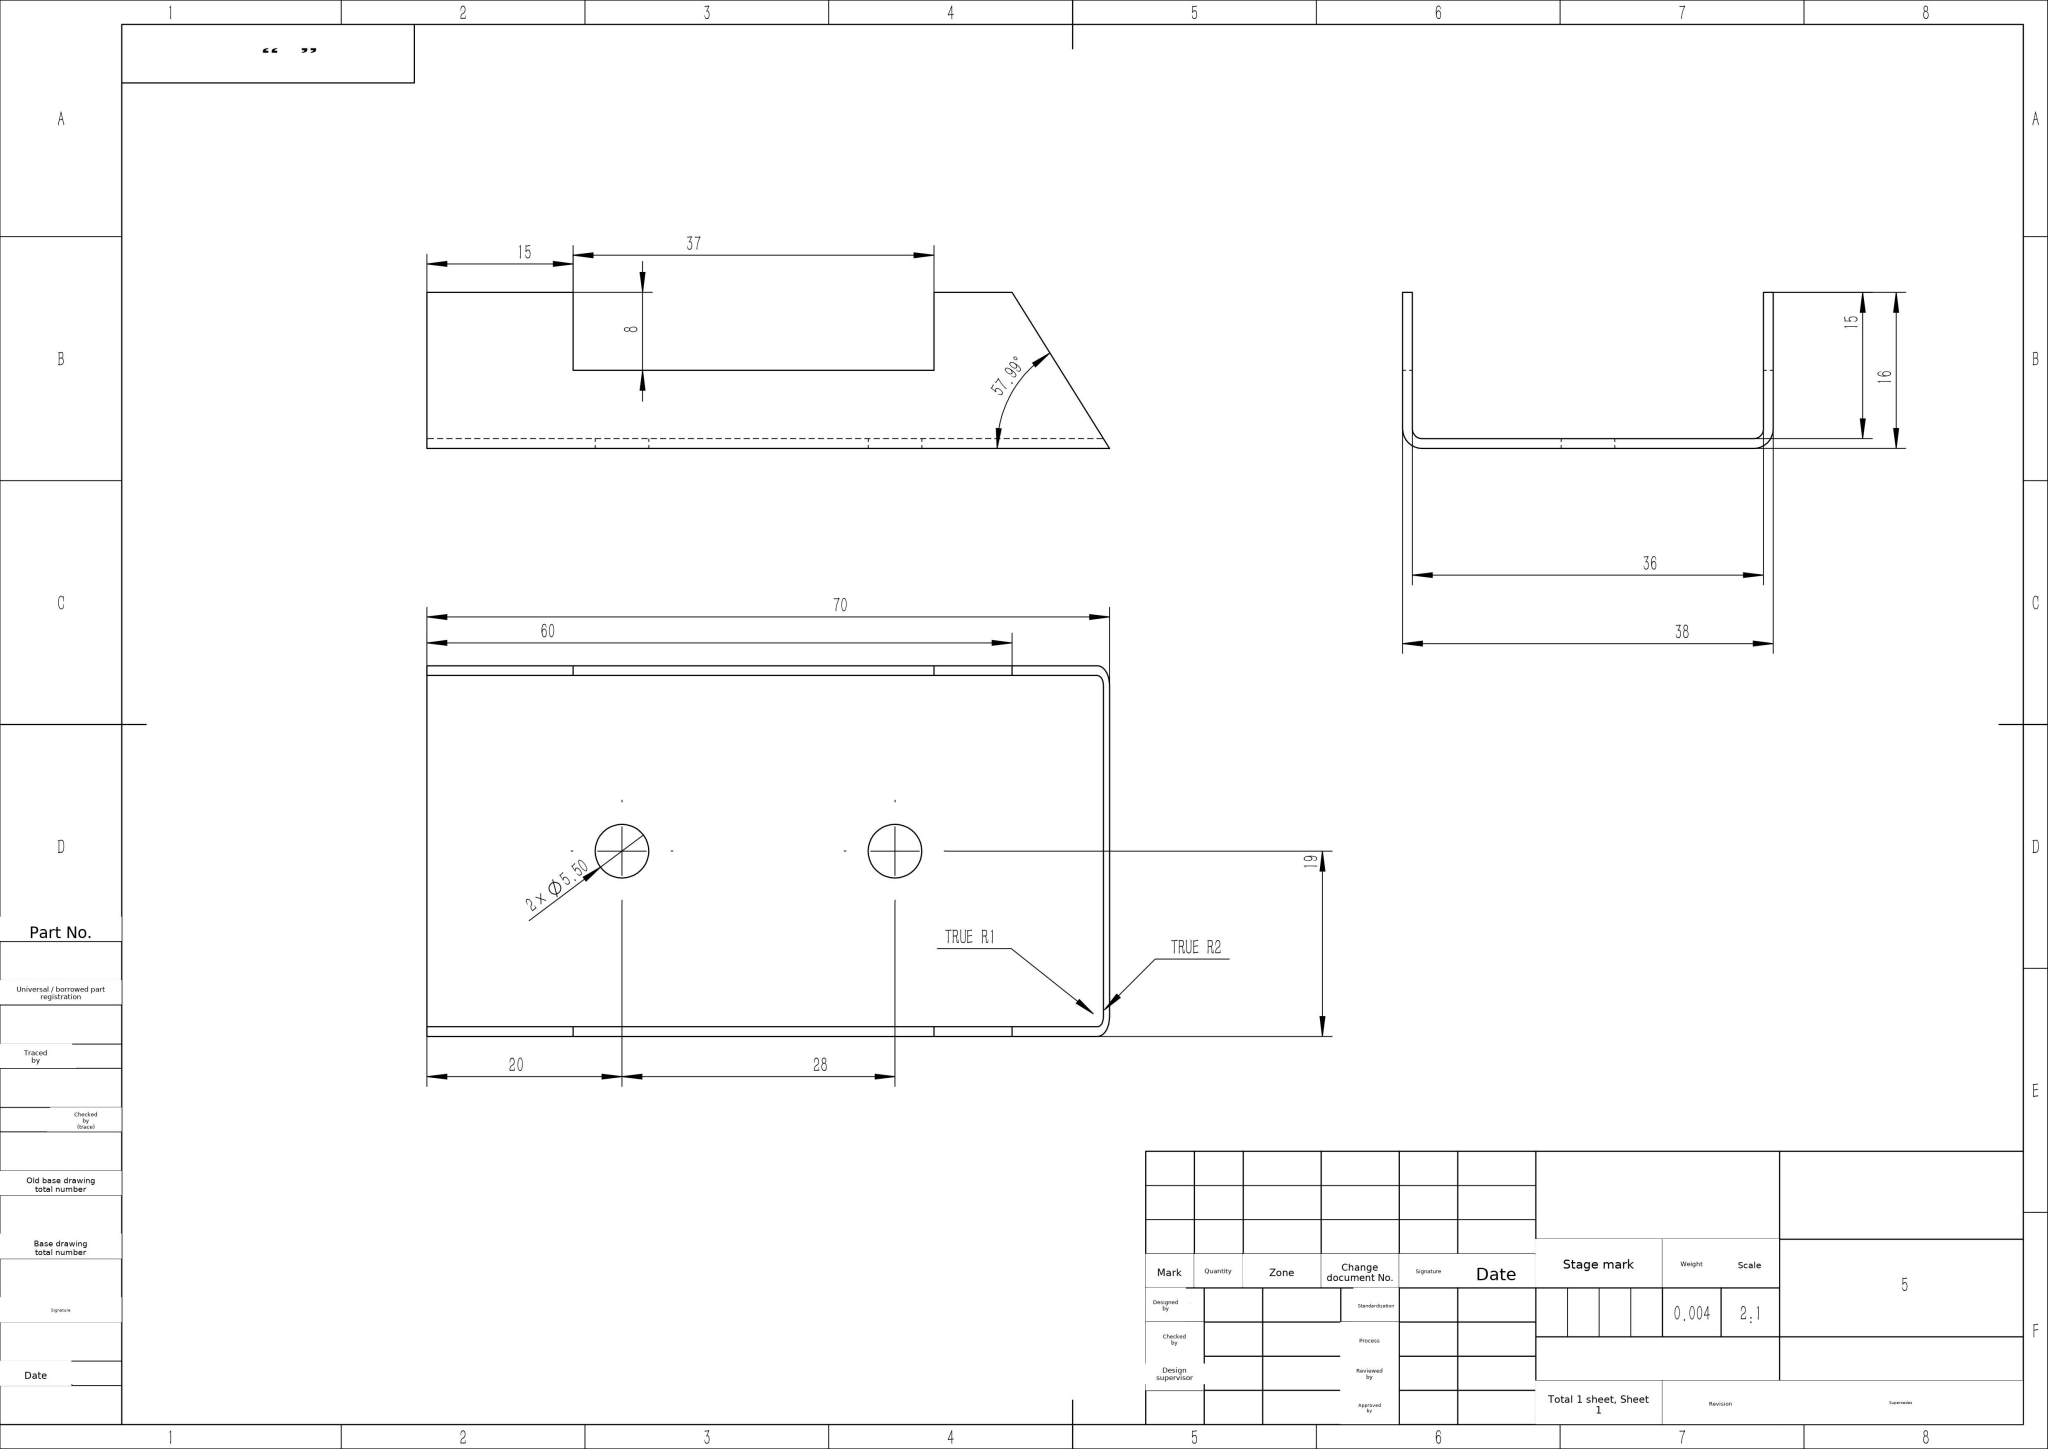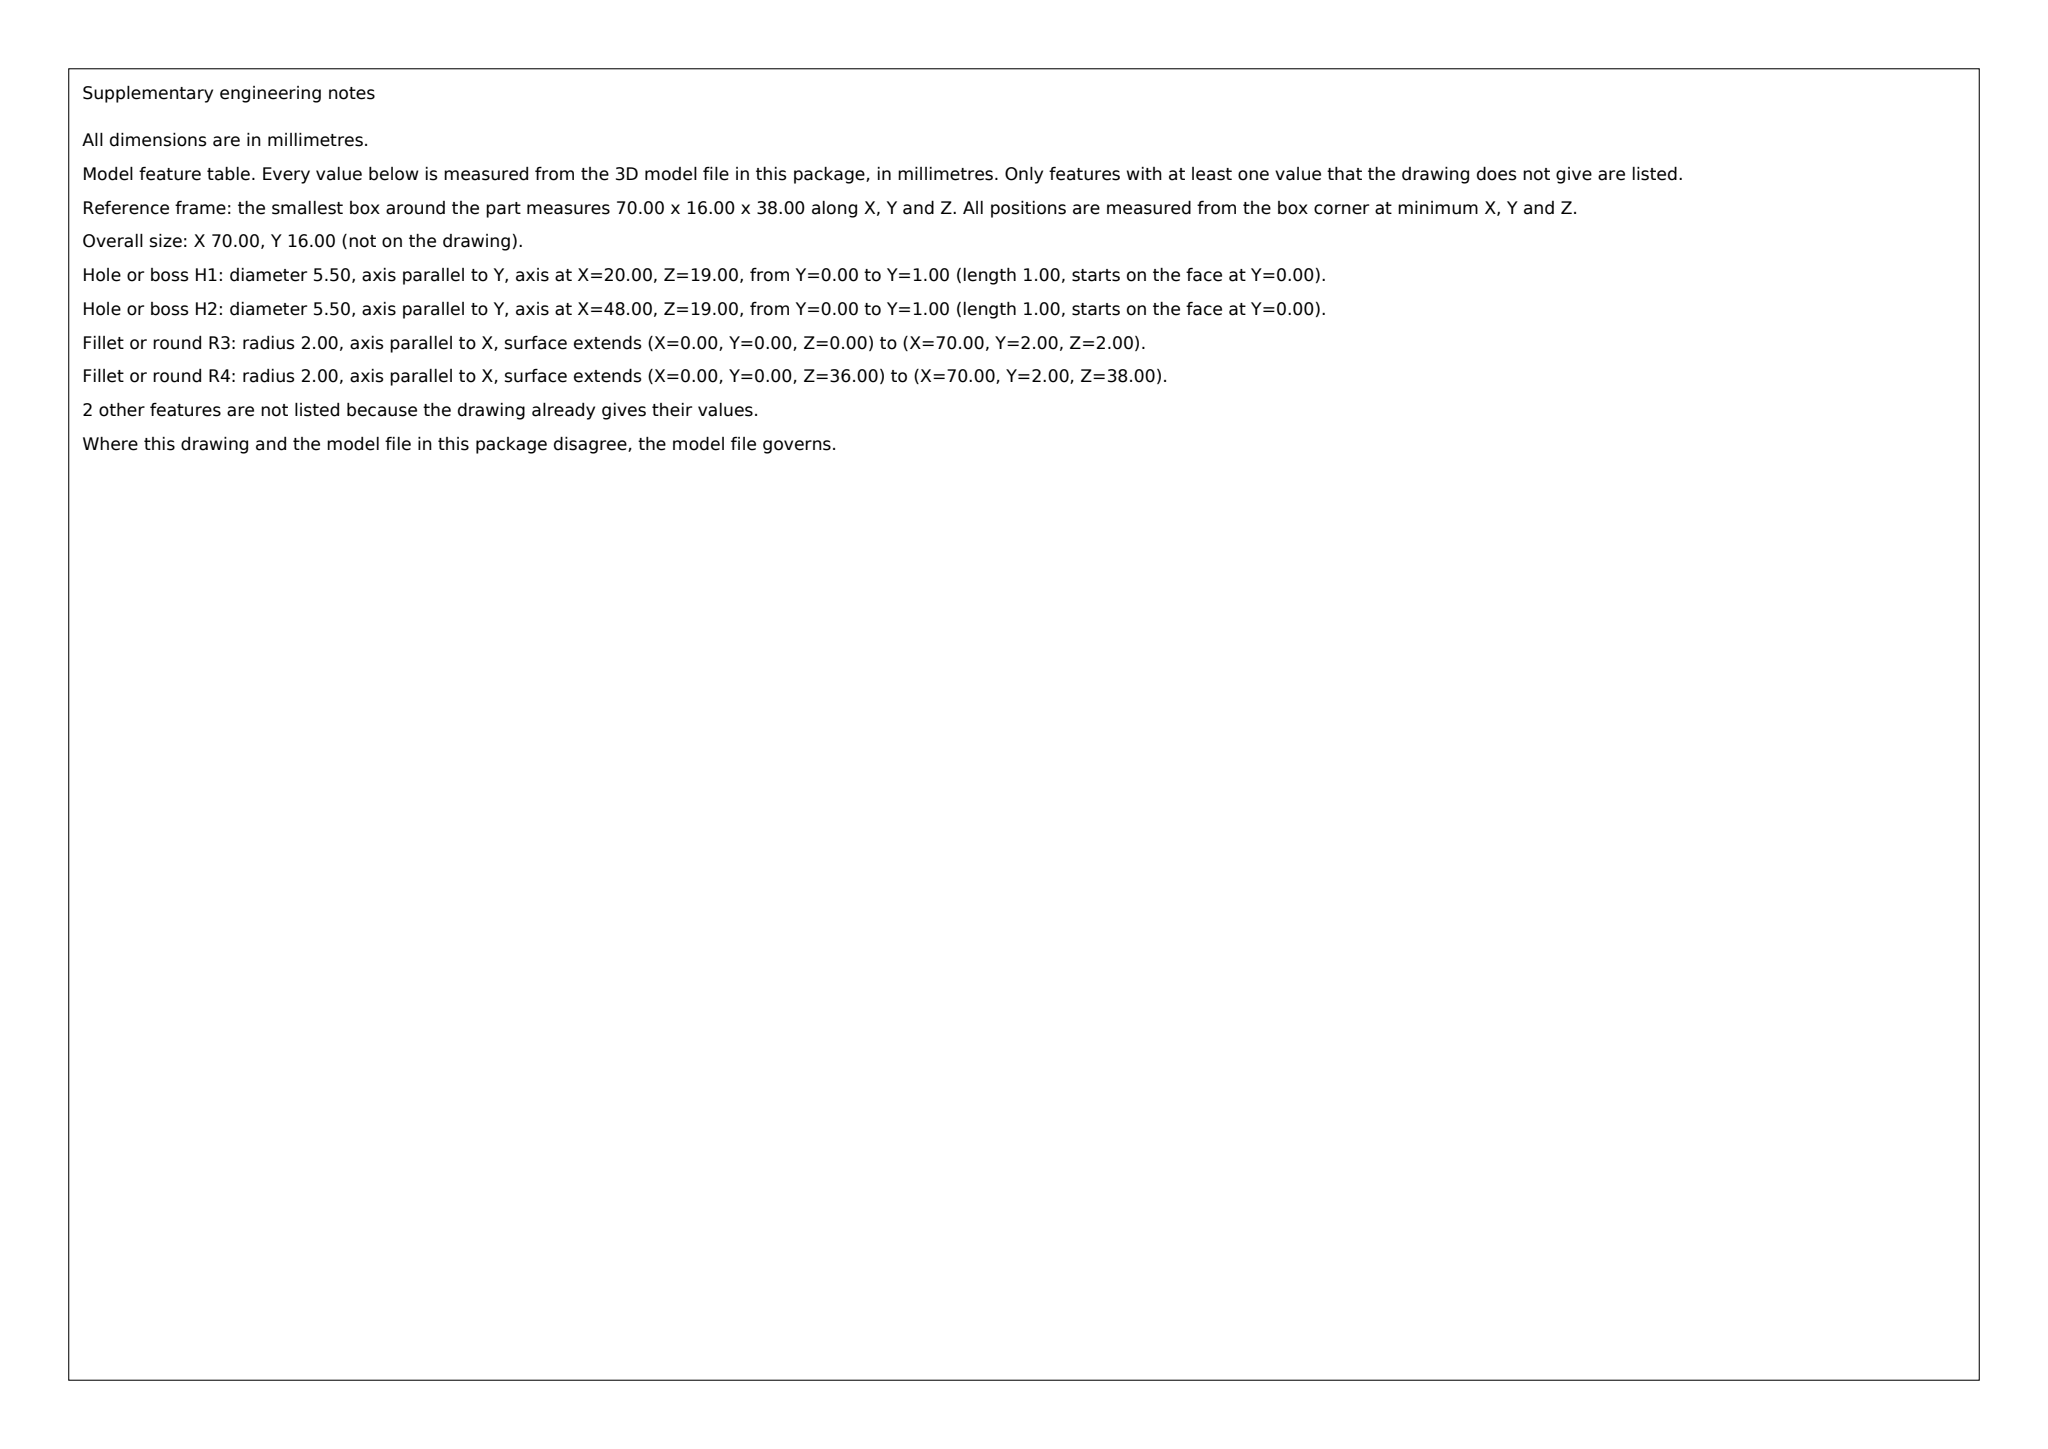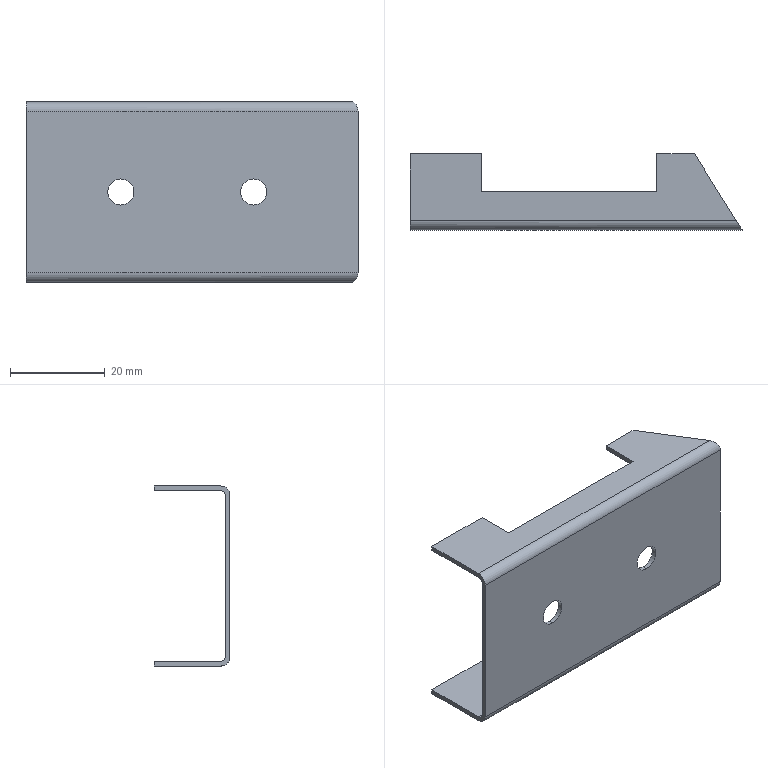Part | SolidWorks | mm | 1 solid | 26 faces | box 70 x 16 x 38 mm | volume 3859 mm3 | plane 18 | cylinder 8 | commonest cylinder face diameters 5.5 x4 2 x2 4 x2
build123d program:
from build123d import *

# Parameters (mm, degrees)
BOSS_EXTRUDE1_DEPTH = 70
FILLET1_R           = 1
FILLET2_R           = 2
SKETCH8_W           = 37
SKETCH8_H           = 9.122
CUT_EXTRUDE1_DEPTH  = 500
CUT_EXTRUDE2_DEPTH  = 500
SKETCH10_R          = 2.75
CUT_EXTRUDE3_DEPTH  = 500


with BuildPart() as part:
    # Sketch1 → Boss-Extrude1 (new body)
    with BuildSketch(Plane(origin=(0, 0, 0), x_dir=(0, 0, -1), z_dir=(1, 0, 0))):
        Polygon((-19, 0), (19, 0), (19, 16), (18, 16), (18, 1), (-18, 1), (-18, 16), (-19, 16), align=None)
    extrude(amount=BOSS_EXTRUDE1_DEPTH)

    # Fillet1
    fillet1_edges = [part.edges().sort_by_distance(p)[0] for p in [
        (35, 1, 18),
        (35, 1, -18),
    ]]
    fillet(fillet1_edges, radius=FILLET1_R)

    # Fillet2
    fillet2_edges = [part.edges().sort_by_distance(p)[0] for p in [
        (35, 0, -19),
        (35, 0, 19),
    ]]
    fillet(fillet2_edges, radius=FILLET2_R)

    # Sketch8 → Cut-Extrude1 (cut, symmetric)
    with BuildSketch(Plane.XY):
        with Locations((33.5, 12.561)):
            Rectangle(SKETCH8_W, SKETCH8_H)
    extrude(amount=CUT_EXTRUDE1_DEPTH, both=True, mode=Mode.SUBTRACT)

    # Sketch9 → Cut-Extrude2 (cut, symmetric)
    with BuildSketch(Plane.XY):
        Polygon((70, 0), (60, 16), (70, 16), align=None)
    extrude(amount=CUT_EXTRUDE2_DEPTH, both=True, mode=Mode.SUBTRACT)

    # Sketch10 → Cut-Extrude3 (cut, symmetric)
    with BuildSketch(Plane(origin=(0, 0, 0), x_dir=(1, 0, 0), z_dir=(0, 1, 0))):
        with Locations(Location((20, 0, 0), (0, 0, 270))):
            Circle(SKETCH10_R)
        with Locations(Location((48, 0, 0), (0, 0, 270))):
            Circle(SKETCH10_R)
    extrude(amount=CUT_EXTRUDE3_DEPTH, both=True, mode=Mode.SUBTRACT)


solid = part.part
STEP:
#1=CARTESIAN_POINT('',(20.,0.,-2.75));
#2=VERTEX_POINT('',#1);
#3=CARTESIAN_POINT('',(20.,-0.,2.75));
#4=VERTEX_POINT('',#3);
#5=CARTESIAN_POINT('',(20.,0.,0.));
#6=DIRECTION('',(0.,1.,0.));
#7=DIRECTION('',(0.,-0.,1.));
#8=AXIS2_PLACEMENT_3D('',#5,#6,#7);
#9=CIRCLE('',#8,2.75);
#10=EDGE_CURVE('',#2,#4,#9,.T.);
#11=ORIENTED_EDGE('',*,*,#10,.F.);
#12=CARTESIAN_POINT('',(20.,1.,-2.75));
#13=VERTEX_POINT('',#12);
#14=CARTESIAN_POINT('',(20.,-500.,-2.75));
#15=DIRECTION('',(0.,1.,0.));
#16=VECTOR('',#15,1000.);
#17=LINE('',#14,#16);
#18=EDGE_CURVE('',#2,#13,#17,.T.);
#19=ORIENTED_EDGE('',*,*,#18,.T.);
#20=CARTESIAN_POINT('',(20.,1.,2.75));
#21=VERTEX_POINT('',#20);
#22=CARTESIAN_POINT('',(20.,1.,0.));
#23=DIRECTION('',(0.,-1.,-0.));
#24=DIRECTION('',(0.,0.,-1.));
#25=AXIS2_PLACEMENT_3D('',#22,#23,#24);
#26=CIRCLE('',#25,2.75);
#27=EDGE_CURVE('',#21,#13,#26,.T.);
#28=ORIENTED_EDGE('',*,*,#27,.F.);
#29=CARTESIAN_POINT('',(20.,-500.,2.75));
#30=DIRECTION('',(0.,1.,0.));
#31=VECTOR('',#30,1000.);
#32=LINE('',#29,#31);
#33=EDGE_CURVE('',#4,#21,#32,.T.);
#34=ORIENTED_EDGE('',*,*,#33,.F.);
#35=EDGE_LOOP('',(#11,#19,#28,#34));
#36=FACE_OUTER_BOUND('',#35,.T.);
#37=CARTESIAN_POINT('',(20.,-500.,0.));
#38=DIRECTION('',(0.,1.,0.));
#39=DIRECTION('',(0.,0.,1.));
#40=AXIS2_PLACEMENT_3D('',#37,#38,#39);
#41=CYLINDRICAL_SURFACE('',#40,2.75);
#42=ADVANCED_FACE('',(#36),#41,.F.);
#43=CARTESIAN_POINT('',(48.,0.,-2.75));
#44=VERTEX_POINT('',#43);
#45=CARTESIAN_POINT('',(48.,-0.,2.75));
#46=VERTEX_POINT('',#45);
#47=CARTESIAN_POINT('',(48.,0.,0.));
#48=DIRECTION('',(0.,1.,0.));
#49=DIRECTION('',(0.,-0.,1.));
#50=AXIS2_PLACEMENT_3D('',#47,#48,#49);
#51=CIRCLE('',#50,2.75);
#52=EDGE_CURVE('',#44,#46,#51,.T.);
#53=ORIENTED_EDGE('',*,*,#52,.F.);
#54=CARTESIAN_POINT('',(48.,1.,-2.75));
#55=VERTEX_POINT('',#54);
#56=CARTESIAN_POINT('',(48.,-500.,-2.75));
#57=DIRECTION('',(0.,1.,0.));
#58=VECTOR('',#57,1000.);
#59=LINE('',#56,#58);
#60=EDGE_CURVE('',#44,#55,#59,.T.);
#61=ORIENTED_EDGE('',*,*,#60,.T.);
#62=CARTESIAN_POINT('',(48.,1.,2.75));
#63=VERTEX_POINT('',#62);
#64=CARTESIAN_POINT('',(48.,1.,0.));
#65=DIRECTION('',(0.,-1.,-0.));
#66=DIRECTION('',(0.,0.,-1.));
#67=AXIS2_PLACEMENT_3D('',#64,#65,#66);
#68=CIRCLE('',#67,2.75);
#69=EDGE_CURVE('',#63,#55,#68,.T.);
#70=ORIENTED_EDGE('',*,*,#69,.F.);
#71=CARTESIAN_POINT('',(48.,-500.,2.75));
#72=DIRECTION('',(0.,1.,0.));
#73=VECTOR('',#72,1000.);
#74=LINE('',#71,#73);
#75=EDGE_CURVE('',#46,#63,#74,.T.);
#76=ORIENTED_EDGE('',*,*,#75,.F.);
#77=EDGE_LOOP('',(#53,#61,#70,#76));
#78=FACE_OUTER_BOUND('',#77,.T.);
#79=CARTESIAN_POINT('',(48.,-500.,0.));
#80=DIRECTION('',(0.,1.,0.));
#81=DIRECTION('',(0.,0.,1.));
#82=AXIS2_PLACEMENT_3D('',#79,#80,#81);
#83=CYLINDRICAL_SURFACE('',#82,2.75);
#84=ADVANCED_FACE('',(#78),#83,.F.);
#85=CARTESIAN_POINT('',(15.,16.,18.));
#86=VERTEX_POINT('',#85);
#87=CARTESIAN_POINT('',(15.,16.,19.));
#88=VERTEX_POINT('',#87);
#89=CARTESIAN_POINT('',(15.,16.,19.));
#90=DIRECTION('',(0.,0.,1.));
#91=VECTOR('',#90,1000.);
#92=LINE('',#89,#91);
#93=EDGE_CURVE('',#86,#88,#92,.T.);
#94=ORIENTED_EDGE('',*,*,#93,.F.);
#95=CARTESIAN_POINT('',(0.,16.,18.));
#96=VERTEX_POINT('',#95);
#97=CARTESIAN_POINT('',(70.,16.,18.));
#98=DIRECTION('',(-1.,0.,0.));
#99=VECTOR('',#98,1000.);
#100=LINE('',#97,#99);
#101=EDGE_CURVE('',#86,#96,#100,.T.);
#102=ORIENTED_EDGE('',*,*,#101,.T.);
#103=CARTESIAN_POINT('',(0.,16.,19.));
#104=VERTEX_POINT('',#103);
#105=CARTESIAN_POINT('',(0.,16.,19.));
#106=DIRECTION('',(0.,0.,-1.));
#107=VECTOR('',#106,1000.);
#108=LINE('',#105,#107);
#109=EDGE_CURVE('',#104,#96,#108,.T.);
#110=ORIENTED_EDGE('',*,*,#109,.F.);
#111=CARTESIAN_POINT('',(70.,16.,19.));
#112=DIRECTION('',(-1.,0.,0.));
#113=VECTOR('',#112,1000.);
#114=LINE('',#111,#113);
#115=EDGE_CURVE('',#88,#104,#114,.T.);
#116=ORIENTED_EDGE('',*,*,#115,.F.);
#117=EDGE_LOOP('',(#94,#102,#110,#116));
#118=FACE_OUTER_BOUND('',#117,.T.);
#119=CARTESIAN_POINT('',(70.,16.,19.));
#120=DIRECTION('',(0.,1.,0.));
#121=DIRECTION('',(0.,0.,1.));
#122=AXIS2_PLACEMENT_3D('',#119,#120,#121);
#123=PLANE('',#122);
#124=ADVANCED_FACE('',(#118),#123,.T.);
#125=CARTESIAN_POINT('',(15.,16.,-18.));
#126=VERTEX_POINT('',#125);
#127=CARTESIAN_POINT('',(0.,16.,-18.));
#128=VERTEX_POINT('',#127);
#129=CARTESIAN_POINT('',(70.,16.,-18.));
#130=DIRECTION('',(-1.,0.,0.));
#131=VECTOR('',#130,1000.);
#132=LINE('',#129,#131);
#133=EDGE_CURVE('',#126,#128,#132,.T.);
#134=ORIENTED_EDGE('',*,*,#133,.F.);
#135=CARTESIAN_POINT('',(15.,16.,-19.));
#136=VERTEX_POINT('',#135);
#137=CARTESIAN_POINT('',(15.,16.,-19.));
#138=DIRECTION('',(0.,0.,-1.));
#139=VECTOR('',#138,1000.);
#140=LINE('',#137,#139);
#141=EDGE_CURVE('',#126,#136,#140,.T.);
#142=ORIENTED_EDGE('',*,*,#141,.T.);
#143=CARTESIAN_POINT('',(0.,16.,-19.));
#144=VERTEX_POINT('',#143);
#145=CARTESIAN_POINT('',(70.,16.,-19.));
#146=DIRECTION('',(-1.,0.,0.));
#147=VECTOR('',#146,1000.);
#148=LINE('',#145,#147);
#149=EDGE_CURVE('',#136,#144,#148,.T.);
#150=ORIENTED_EDGE('',*,*,#149,.T.);
#151=CARTESIAN_POINT('',(0.,16.,-19.));
#152=DIRECTION('',(0.,0.,1.));
#153=VECTOR('',#152,1000.);
#154=LINE('',#151,#153);
#155=EDGE_CURVE('',#144,#128,#154,.T.);
#156=ORIENTED_EDGE('',*,*,#155,.T.);
#157=EDGE_LOOP('',(#134,#142,#150,#156));
#158=FACE_OUTER_BOUND('',#157,.T.);
#159=CARTESIAN_POINT('',(70.,16.,-19.));
#160=DIRECTION('',(0.,-1.,0.));
#161=DIRECTION('',(0.,0.,-1.));
#162=AXIS2_PLACEMENT_3D('',#159,#160,#161);
#163=PLANE('',#162);
#164=ADVANCED_FACE('',(#158),#163,.F.);
#165=CARTESIAN_POINT('',(0.,2.,-18.));
#166=VERTEX_POINT('',#165);
#167=CARTESIAN_POINT('',(68.75,2.,-18.));
#168=VERTEX_POINT('',#167);
#169=CARTESIAN_POINT('',(70.,2.,-18.));
#170=DIRECTION('',(1.,0.,0.));
#171=VECTOR('',#170,1000.);
#172=LINE('',#169,#171);
#173=EDGE_CURVE('',#166,#168,#172,.T.);
#174=ORIENTED_EDGE('',*,*,#173,.T.);
#175=CARTESIAN_POINT('',(60.,16.,-18.));
#176=VERTEX_POINT('',#175);
#177=CARTESIAN_POINT('',(62.809,11.506,-18.));
#178=DIRECTION('',(-0.53,0.848,0.));
#179=VECTOR('',#178,1000.);
#180=LINE('',#177,#179);
#181=EDGE_CURVE('',#168,#176,#180,.T.);
#182=ORIENTED_EDGE('',*,*,#181,.T.);
#183=CARTESIAN_POINT('',(52.,16.,-18.));
#184=VERTEX_POINT('',#183);
#185=CARTESIAN_POINT('',(70.,16.,-18.));
#186=DIRECTION('',(-1.,0.,0.));
#187=VECTOR('',#186,1000.);
#188=LINE('',#185,#187);
#189=EDGE_CURVE('',#176,#184,#188,.T.);
#190=ORIENTED_EDGE('',*,*,#189,.T.);
#191=CARTESIAN_POINT('',(52.,8.,-18.));
#192=VERTEX_POINT('',#191);
#193=CARTESIAN_POINT('',(52.,16.,-18.));
#194=DIRECTION('',(0.,-1.,-0.));
#195=VECTOR('',#194,1000.);
#196=LINE('',#193,#195);
#197=EDGE_CURVE('',#184,#192,#196,.T.);
#198=ORIENTED_EDGE('',*,*,#197,.T.);
#199=CARTESIAN_POINT('',(15.,8.,-18.));
#200=VERTEX_POINT('',#199);
#201=CARTESIAN_POINT('',(70.,8.,-18.));
#202=DIRECTION('',(-1.,0.,0.));
#203=VECTOR('',#202,1000.);
#204=LINE('',#201,#203);
#205=EDGE_CURVE('',#192,#200,#204,.T.);
#206=ORIENTED_EDGE('',*,*,#205,.T.);
#207=CARTESIAN_POINT('',(15.,16.,-18.));
#208=DIRECTION('',(0.,1.,0.));
#209=VECTOR('',#208,1000.);
#210=LINE('',#207,#209);
#211=EDGE_CURVE('',#200,#126,#210,.T.);
#212=ORIENTED_EDGE('',*,*,#211,.T.);
#213=ORIENTED_EDGE('',*,*,#133,.T.);
#214=CARTESIAN_POINT('',(0.,16.,-18.));
#215=DIRECTION('',(0.,-1.,-0.));
#216=VECTOR('',#215,1000.);
#217=LINE('',#214,#216);
#218=EDGE_CURVE('',#128,#166,#217,.T.);
#219=ORIENTED_EDGE('',*,*,#218,.T.);
#220=EDGE_LOOP('',(#174,#182,#190,#198,#206,#212,#213,#219));
#221=FACE_OUTER_BOUND('',#220,.T.);
#222=CARTESIAN_POINT('',(70.,16.,-18.));
#223=DIRECTION('',(0.,0.,-1.));
#224=DIRECTION('',(0.,1.,0.));
#225=AXIS2_PLACEMENT_3D('',#222,#223,#224);
#226=PLANE('',#225);
#227=ADVANCED_FACE('',(#221),#226,.F.);
#228=ORIENTED_EDGE('',*,*,#27,.T.);
#229=CARTESIAN_POINT('',(20.,1.,0.));
#230=DIRECTION('',(0.,-1.,-0.));
#231=DIRECTION('',(0.,0.,-1.));
#232=AXIS2_PLACEMENT_3D('',#229,#230,#231);
#233=CIRCLE('',#232,2.75);
#234=EDGE_CURVE('',#13,#21,#233,.T.);
#235=ORIENTED_EDGE('',*,*,#234,.T.);
#236=EDGE_LOOP('',(#228,#235));
#237=FACE_BOUND('',#236,.T.);
#238=ORIENTED_EDGE('',*,*,#69,.T.);
#239=CARTESIAN_POINT('',(48.,1.,0.));
#240=DIRECTION('',(0.,-1.,-0.));
#241=DIRECTION('',(0.,0.,-1.));
#242=AXIS2_PLACEMENT_3D('',#239,#240,#241);
#243=CIRCLE('',#242,2.75);
#244=EDGE_CURVE('',#55,#63,#243,.T.);
#245=ORIENTED_EDGE('',*,*,#244,.T.);
#246=EDGE_LOOP('',(#238,#245));
#247=FACE_BOUND('',#246,.T.);
#248=CARTESIAN_POINT('',(0.,1.,17.));
#249=VERTEX_POINT('',#248);
#250=CARTESIAN_POINT('',(69.375,1.,17.));
#251=VERTEX_POINT('',#250);
#252=CARTESIAN_POINT('',(70.,1.,17.));
#253=DIRECTION('',(1.,0.,0.));
#254=VECTOR('',#253,1000.);
#255=LINE('',#252,#254);
#256=EDGE_CURVE('',#249,#251,#255,.T.);
#257=ORIENTED_EDGE('',*,*,#256,.T.);
#258=CARTESIAN_POINT('',(69.375,1.,-17.));
#259=VERTEX_POINT('',#258);
#260=CARTESIAN_POINT('',(69.375,1.,-18.));
#261=DIRECTION('',(-0.,0.,-1.));
#262=VECTOR('',#261,1000.);
#263=LINE('',#260,#262);
#264=EDGE_CURVE('',#251,#259,#263,.T.);
#265=ORIENTED_EDGE('',*,*,#264,.T.);
#266=CARTESIAN_POINT('',(0.,1.,-17.));
#267=VERTEX_POINT('',#266);
#268=CARTESIAN_POINT('',(0.,1.,-17.));
#269=DIRECTION('',(-1.,0.,0.));
#270=VECTOR('',#269,1000.);
#271=LINE('',#268,#270);
#272=EDGE_CURVE('',#259,#267,#271,.T.);
#273=ORIENTED_EDGE('',*,*,#272,.T.);
#274=CARTESIAN_POINT('',(0.,1.,-18.));
#275=DIRECTION('',(0.,-0.,1.));
#276=VECTOR('',#275,1000.);
#277=LINE('',#274,#276);
#278=EDGE_CURVE('',#267,#249,#277,.T.);
#279=ORIENTED_EDGE('',*,*,#278,.T.);
#280=EDGE_LOOP('',(#257,#265,#273,#279));
#281=FACE_OUTER_BOUND('',#280,.T.);
#282=CARTESIAN_POINT('',(70.,1.,-18.));
#283=DIRECTION('',(0.,-1.,-0.));
#284=DIRECTION('',(0.,0.,-1.));
#285=AXIS2_PLACEMENT_3D('',#282,#283,#284);
#286=PLANE('',#285);
#287=ADVANCED_FACE('',(#237,#247,#281),#286,.F.);
#288=CARTESIAN_POINT('',(68.75,2.,18.));
#289=VERTEX_POINT('',#288);
#290=CARTESIAN_POINT('',(60.,16.,18.));
#291=VERTEX_POINT('',#290);
#292=CARTESIAN_POINT('',(62.809,11.506,18.));
#293=DIRECTION('',(-0.53,0.848,0.));
#294=VECTOR('',#293,1000.);
#295=LINE('',#292,#294);
#296=EDGE_CURVE('',#289,#291,#295,.T.);
#297=ORIENTED_EDGE('',*,*,#296,.F.);
#298=CARTESIAN_POINT('',(0.,2.,18.));
#299=VERTEX_POINT('',#298);
#300=CARTESIAN_POINT('',(70.,2.,18.));
#301=DIRECTION('',(-1.,0.,0.));
#302=VECTOR('',#301,1000.);
#303=LINE('',#300,#302);
#304=EDGE_CURVE('',#289,#299,#303,.T.);
#305=ORIENTED_EDGE('',*,*,#304,.T.);
#306=CARTESIAN_POINT('',(0.,16.,18.));
#307=DIRECTION('',(0.,-1.,-0.));
#308=VECTOR('',#307,1000.);
#309=LINE('',#306,#308);
#310=EDGE_CURVE('',#96,#299,#309,.T.);
#311=ORIENTED_EDGE('',*,*,#310,.F.);
#312=ORIENTED_EDGE('',*,*,#101,.F.);
#313=CARTESIAN_POINT('',(15.,8.,18.));
#314=VERTEX_POINT('',#313);
#315=CARTESIAN_POINT('',(15.,16.,18.));
#316=DIRECTION('',(0.,1.,0.));
#317=VECTOR('',#316,1000.);
#318=LINE('',#315,#317);
#319=EDGE_CURVE('',#314,#86,#318,.T.);
#320=ORIENTED_EDGE('',*,*,#319,.F.);
#321=CARTESIAN_POINT('',(52.,8.,18.));
#322=VERTEX_POINT('',#321);
#323=CARTESIAN_POINT('',(70.,8.,18.));
#324=DIRECTION('',(-1.,0.,0.));
#325=VECTOR('',#324,1000.);
#326=LINE('',#323,#325);
#327=EDGE_CURVE('',#322,#314,#326,.T.);
#328=ORIENTED_EDGE('',*,*,#327,.F.);
#329=CARTESIAN_POINT('',(52.,16.,18.));
#330=VERTEX_POINT('',#329);
#331=CARTESIAN_POINT('',(52.,16.,18.));
#332=DIRECTION('',(0.,-1.,-0.));
#333=VECTOR('',#332,1000.);
#334=LINE('',#331,#333);
#335=EDGE_CURVE('',#330,#322,#334,.T.);
#336=ORIENTED_EDGE('',*,*,#335,.F.);
#337=CARTESIAN_POINT('',(70.,16.,18.));
#338=DIRECTION('',(-1.,0.,0.));
#339=VECTOR('',#338,1000.);
#340=LINE('',#337,#339);
#341=EDGE_CURVE('',#291,#330,#340,.T.);
#342=ORIENTED_EDGE('',*,*,#341,.F.);
#343=EDGE_LOOP('',(#297,#305,#311,#312,#320,#328,#336,#342));
#344=FACE_OUTER_BOUND('',#343,.T.);
#345=CARTESIAN_POINT('',(70.,16.,18.));
#346=DIRECTION('',(0.,0.,-1.));
#347=DIRECTION('',(0.,1.,0.));
#348=AXIS2_PLACEMENT_3D('',#345,#346,#347);
#349=PLANE('',#348);
#350=ADVANCED_FACE('',(#344),#349,.T.);
#351=CARTESIAN_POINT('',(60.,16.,19.));
#352=VERTEX_POINT('',#351);
#353=CARTESIAN_POINT('',(60.,16.,-500.));
#354=DIRECTION('',(0.,0.,1.));
#355=VECTOR('',#354,1000.);
#356=LINE('',#353,#355);
#357=EDGE_CURVE('',#291,#352,#356,.T.);
#358=ORIENTED_EDGE('',*,*,#357,.F.);
#359=ORIENTED_EDGE('',*,*,#341,.T.);
#360=CARTESIAN_POINT('',(52.,16.,19.));
#361=VERTEX_POINT('',#360);
#362=CARTESIAN_POINT('',(52.,16.,19.));
#363=DIRECTION('',(0.,0.,-1.));
#364=VECTOR('',#363,1000.);
#365=LINE('',#362,#364);
#366=EDGE_CURVE('',#361,#330,#365,.T.);
#367=ORIENTED_EDGE('',*,*,#366,.F.);
#368=CARTESIAN_POINT('',(70.,16.,19.));
#369=DIRECTION('',(-1.,0.,0.));
#370=VECTOR('',#369,1000.);
#371=LINE('',#368,#370);
#372=EDGE_CURVE('',#352,#361,#371,.T.);
#373=ORIENTED_EDGE('',*,*,#372,.F.);
#374=EDGE_LOOP('',(#358,#359,#367,#373));
#375=FACE_OUTER_BOUND('',#374,.T.);
#376=CARTESIAN_POINT('',(70.,16.,19.));
#377=DIRECTION('',(0.,1.,0.));
#378=DIRECTION('',(0.,0.,1.));
#379=AXIS2_PLACEMENT_3D('',#376,#377,#378);
#380=PLANE('',#379);
#381=ADVANCED_FACE('',(#375),#380,.T.);
#382=CARTESIAN_POINT('',(68.75,2.,19.));
#383=VERTEX_POINT('',#382);
#384=CARTESIAN_POINT('',(70.,0.,19.));
#385=DIRECTION('',(0.53,-0.848,-0.));
#386=VECTOR('',#385,1000.);
#387=LINE('',#384,#386);
#388=EDGE_CURVE('',#352,#383,#387,.T.);
#389=ORIENTED_EDGE('',*,*,#388,.F.);
#390=ORIENTED_EDGE('',*,*,#372,.T.);
#391=CARTESIAN_POINT('',(52.,8.,19.));
#392=VERTEX_POINT('',#391);
#393=CARTESIAN_POINT('',(52.,0.,19.));
#394=DIRECTION('',(0.,1.,0.));
#395=VECTOR('',#394,1000.);
#396=LINE('',#393,#395);
#397=EDGE_CURVE('',#392,#361,#396,.T.);
#398=ORIENTED_EDGE('',*,*,#397,.F.);
#399=CARTESIAN_POINT('',(15.,8.,19.));
#400=VERTEX_POINT('',#399);
#401=CARTESIAN_POINT('',(70.,8.,19.));
#402=DIRECTION('',(1.,0.,0.));
#403=VECTOR('',#402,1000.);
#404=LINE('',#401,#403);
#405=EDGE_CURVE('',#400,#392,#404,.T.);
#406=ORIENTED_EDGE('',*,*,#405,.F.);
#407=CARTESIAN_POINT('',(15.,0.,19.));
#408=DIRECTION('',(0.,-1.,-0.));
#409=VECTOR('',#408,1000.);
#410=LINE('',#407,#409);
#411=EDGE_CURVE('',#88,#400,#410,.T.);
#412=ORIENTED_EDGE('',*,*,#411,.F.);
#413=ORIENTED_EDGE('',*,*,#115,.T.);
#414=CARTESIAN_POINT('',(0.,2.,19.));
#415=VERTEX_POINT('',#414);
#416=CARTESIAN_POINT('',(0.,0.,19.));
#417=DIRECTION('',(0.,1.,0.));
#418=VECTOR('',#417,1000.);
#419=LINE('',#416,#418);
#420=EDGE_CURVE('',#415,#104,#419,.T.);
#421=ORIENTED_EDGE('',*,*,#420,.F.);
#422=CARTESIAN_POINT('',(70.,2.,19.));
#423=DIRECTION('',(1.,0.,0.));
#424=VECTOR('',#423,1000.);
#425=LINE('',#422,#424);
#426=EDGE_CURVE('',#415,#383,#425,.T.);
#427=ORIENTED_EDGE('',*,*,#426,.T.);
#428=EDGE_LOOP('',(#389,#390,#398,#406,#412,#413,#421,#427));
#429=FACE_OUTER_BOUND('',#428,.T.);
#430=CARTESIAN_POINT('',(70.,0.,19.));
#431=DIRECTION('',(0.,-0.,1.));
#432=DIRECTION('',(0.,-1.,-0.));
#433=AXIS2_PLACEMENT_3D('',#430,#431,#432);
#434=PLANE('',#433);
#435=ADVANCED_FACE('',(#429),#434,.T.);
#436=CARTESIAN_POINT('',(20.,0.,0.));
#437=DIRECTION('',(0.,1.,0.));
#438=DIRECTION('',(0.,-0.,1.));
#439=AXIS2_PLACEMENT_3D('',#436,#437,#438);
#440=CIRCLE('',#439,2.75);
#441=EDGE_CURVE('',#4,#2,#440,.T.);
#442=ORIENTED_EDGE('',*,*,#441,.T.);
#443=ORIENTED_EDGE('',*,*,#10,.T.);
#444=EDGE_LOOP('',(#442,#443));
#445=FACE_BOUND('',#444,.T.);
#446=CARTESIAN_POINT('',(48.,0.,0.));
#447=DIRECTION('',(0.,1.,0.));
#448=DIRECTION('',(0.,-0.,1.));
#449=AXIS2_PLACEMENT_3D('',#446,#447,#448);
#450=CIRCLE('',#449,2.75);
#451=EDGE_CURVE('',#46,#44,#450,.T.);
#452=ORIENTED_EDGE('',*,*,#451,.T.);
#453=ORIENTED_EDGE('',*,*,#52,.T.);
#454=EDGE_LOOP('',(#452,#453));
#455=FACE_BOUND('',#454,.T.);
#456=CARTESIAN_POINT('',(70.,0.,17.));
#457=VERTEX_POINT('',#456);
#458=CARTESIAN_POINT('',(70.,0.,-17.));
#459=VERTEX_POINT('',#458);
#460=CARTESIAN_POINT('',(70.,0.,19.));
#461=DIRECTION('',(0.,0.,-1.));
#462=VECTOR('',#461,1000.);
#463=LINE('',#460,#462);
#464=EDGE_CURVE('',#457,#459,#463,.T.);
#465=ORIENTED_EDGE('',*,*,#464,.F.);
#466=CARTESIAN_POINT('',(0.,0.,17.));
#467=VERTEX_POINT('',#466);
#468=CARTESIAN_POINT('',(0.,0.,17.));
#469=DIRECTION('',(-1.,0.,0.));
#470=VECTOR('',#469,1000.);
#471=LINE('',#468,#470);
#472=EDGE_CURVE('',#457,#467,#471,.T.);
#473=ORIENTED_EDGE('',*,*,#472,.T.);
#474=CARTESIAN_POINT('',(0.,0.,-17.));
#475=VERTEX_POINT('',#474);
#476=CARTESIAN_POINT('',(0.,0.,19.));
#477=DIRECTION('',(0.,0.,-1.));
#478=VECTOR('',#477,1000.);
#479=LINE('',#476,#478);
#480=EDGE_CURVE('',#467,#475,#479,.T.);
#481=ORIENTED_EDGE('',*,*,#480,.T.);
#482=CARTESIAN_POINT('',(70.,0.,-17.));
#483=DIRECTION('',(1.,0.,0.));
#484=VECTOR('',#483,1000.);
#485=LINE('',#482,#484);
#486=EDGE_CURVE('',#475,#459,#485,.T.);
#487=ORIENTED_EDGE('',*,*,#486,.T.);
#488=EDGE_LOOP('',(#465,#473,#481,#487));
#489=FACE_OUTER_BOUND('',#488,.T.);
#490=CARTESIAN_POINT('',(70.,0.,19.));
#491=DIRECTION('',(0.,1.,0.));
#492=DIRECTION('',(0.,-0.,1.));
#493=AXIS2_PLACEMENT_3D('',#490,#491,#492);
#494=PLANE('',#493);
#495=ADVANCED_FACE('',(#445,#455,#489),#494,.F.);
#496=CARTESIAN_POINT('',(60.,16.,-19.));
#497=VERTEX_POINT('',#496);
#498=CARTESIAN_POINT('',(52.,16.,-19.));
#499=VERTEX_POINT('',#498);
#500=CARTESIAN_POINT('',(70.,16.,-19.));
#501=DIRECTION('',(-1.,0.,0.));
#502=VECTOR('',#501,1000.);
#503=LINE('',#500,#502);
#504=EDGE_CURVE('',#497,#499,#503,.T.);
#505=ORIENTED_EDGE('',*,*,#504,.F.);
#506=CARTESIAN_POINT('',(68.75,2.,-19.));
#507=VERTEX_POINT('',#506);
#508=CARTESIAN_POINT('',(70.,0.,-19.));
#509=DIRECTION('',(0.53,-0.848,-0.));
#510=VECTOR('',#509,1000.);
#511=LINE('',#508,#510);
#512=EDGE_CURVE('',#497,#507,#511,.T.);
#513=ORIENTED_EDGE('',*,*,#512,.T.);
#514=CARTESIAN_POINT('',(0.,2.,-19.));
#515=VERTEX_POINT('',#514);
#516=CARTESIAN_POINT('',(70.,2.,-19.));
#517=DIRECTION('',(-1.,0.,0.));
#518=VECTOR('',#517,1000.);
#519=LINE('',#516,#518);
#520=EDGE_CURVE('',#507,#515,#519,.T.);
#521=ORIENTED_EDGE('',*,*,#520,.T.);
#522=CARTESIAN_POINT('',(0.,0.,-19.));
#523=DIRECTION('',(0.,1.,0.));
#524=VECTOR('',#523,1000.);
#525=LINE('',#522,#524);
#526=EDGE_CURVE('',#515,#144,#525,.T.);
#527=ORIENTED_EDGE('',*,*,#526,.T.);
#528=ORIENTED_EDGE('',*,*,#149,.F.);
#529=CARTESIAN_POINT('',(15.,8.,-19.));
#530=VERTEX_POINT('',#529);
#531=CARTESIAN_POINT('',(15.,0.,-19.));
#532=DIRECTION('',(0.,-1.,-0.));
#533=VECTOR('',#532,1000.);
#534=LINE('',#531,#533);
#535=EDGE_CURVE('',#136,#530,#534,.T.);
#536=ORIENTED_EDGE('',*,*,#535,.T.);
#537=CARTESIAN_POINT('',(52.,8.,-19.));
#538=VERTEX_POINT('',#537);
#539=CARTESIAN_POINT('',(70.,8.,-19.));
#540=DIRECTION('',(1.,0.,0.));
#541=VECTOR('',#540,1000.);
#542=LINE('',#539,#541);
#543=EDGE_CURVE('',#530,#538,#542,.T.);
#544=ORIENTED_EDGE('',*,*,#543,.T.);
#545=CARTESIAN_POINT('',(52.,0.,-19.));
#546=DIRECTION('',(0.,1.,0.));
#547=VECTOR('',#546,1000.);
#548=LINE('',#545,#547);
#549=EDGE_CURVE('',#538,#499,#548,.T.);
#550=ORIENTED_EDGE('',*,*,#549,.T.);
#551=EDGE_LOOP('',(#505,#513,#521,#527,#528,#536,#544,#550));
#552=FACE_OUTER_BOUND('',#551,.T.);
#553=CARTESIAN_POINT('',(70.,0.,-19.));
#554=DIRECTION('',(0.,-0.,1.));
#555=DIRECTION('',(0.,-1.,-0.));
#556=AXIS2_PLACEMENT_3D('',#553,#554,#555);
#557=PLANE('',#556);
#558=ADVANCED_FACE('',(#552),#557,.F.);
#559=ORIENTED_EDGE('',*,*,#189,.F.);
#560=CARTESIAN_POINT('',(60.,16.,-500.));
#561=DIRECTION('',(0.,0.,1.));
#562=VECTOR('',#561,1000.);
#563=LINE('',#560,#562);
#564=EDGE_CURVE('',#497,#176,#563,.T.);
#565=ORIENTED_EDGE('',*,*,#564,.F.);
#566=ORIENTED_EDGE('',*,*,#504,.T.);
#567=CARTESIAN_POINT('',(52.,16.,-19.));
#568=DIRECTION('',(0.,0.,1.));
#569=VECTOR('',#568,1000.);
#570=LINE('',#567,#569);
#571=EDGE_CURVE('',#499,#184,#570,.T.);
#572=ORIENTED_EDGE('',*,*,#571,.T.);
#573=EDGE_LOOP('',(#559,#565,#566,#572));
#574=FACE_OUTER_BOUND('',#573,.T.);
#575=CARTESIAN_POINT('',(70.,16.,-19.));
#576=DIRECTION('',(0.,-1.,0.));
#577=DIRECTION('',(0.,0.,-1.));
#578=AXIS2_PLACEMENT_3D('',#575,#576,#577);
#579=PLANE('',#578);
#580=ADVANCED_FACE('',(#574),#579,.F.);
#581=ORIENTED_EDGE('',*,*,#480,.F.);
#582=CARTESIAN_POINT('',(0.,2.,17.));
#583=DIRECTION('',(-1.,0.,0.));
#584=DIRECTION('',(0.,0.,1.));
#585=AXIS2_PLACEMENT_3D('',#582,#583,#584);
#586=CIRCLE('',#585,2.);
#587=EDGE_CURVE('',#467,#415,#586,.T.);
#588=ORIENTED_EDGE('',*,*,#587,.T.);
#589=ORIENTED_EDGE('',*,*,#420,.T.);
#590=ORIENTED_EDGE('',*,*,#109,.T.);
#591=ORIENTED_EDGE('',*,*,#310,.T.);
#592=CARTESIAN_POINT('',(0.,2.,17.));
#593=DIRECTION('',(1.,0.,0.));
#594=DIRECTION('',(0.,0.,1.));
#595=AXIS2_PLACEMENT_3D('',#592,#593,#594);
#596=CIRCLE('',#595,1.);
#597=EDGE_CURVE('',#299,#249,#596,.T.);
#598=ORIENTED_EDGE('',*,*,#597,.T.);
#599=ORIENTED_EDGE('',*,*,#278,.F.);
#600=CARTESIAN_POINT('',(0.,2.,-17.));
#601=DIRECTION('',(1.,0.,0.));
#602=DIRECTION('',(0.,0.,1.));
#603=AXIS2_PLACEMENT_3D('',#600,#601,#602);
#604=CIRCLE('',#603,1.);
#605=EDGE_CURVE('',#267,#166,#604,.T.);
#606=ORIENTED_EDGE('',*,*,#605,.T.);
#607=ORIENTED_EDGE('',*,*,#218,.F.);
#608=ORIENTED_EDGE('',*,*,#155,.F.);
#609=ORIENTED_EDGE('',*,*,#526,.F.);
#610=CARTESIAN_POINT('',(0.,2.,-17.));
#611=DIRECTION('',(-1.,0.,0.));
#612=DIRECTION('',(0.,0.,1.));
#613=AXIS2_PLACEMENT_3D('',#610,#611,#612);
#614=CIRCLE('',#613,2.);
#615=EDGE_CURVE('',#515,#475,#614,.T.);
#616=ORIENTED_EDGE('',*,*,#615,.T.);
#617=EDGE_LOOP('',(#581,#588,#589,#590,#591,#598,#599,#606,#607,#608,#609,#616));
#618=FACE_OUTER_BOUND('',#617,.T.);
#619=CARTESIAN_POINT('',(0.,0.,0.));
#620=DIRECTION('',(-1.,0.,0.));
#621=DIRECTION('',(0.,0.,1.));
#622=AXIS2_PLACEMENT_3D('',#619,#620,#621);
#623=PLANE('',#622);
#624=ADVANCED_FACE('',(#618),#623,.T.);
#625=ORIENTED_EDGE('',*,*,#304,.F.);
#626=CARTESIAN_POINT('',(68.75,2.,18.));
#627=CARTESIAN_POINT('',(69.116,1.414,18.));
#628=CARTESIAN_POINT('',(69.375,1.,17.586));
#629=CARTESIAN_POINT('',(69.375,1.,17.));
#630=(BOUNDED_CURVE()B_SPLINE_CURVE(3,(#626,#627,#628,#629),.UNSPECIFIED.,.F.,.T.)B_SPLINE_CURVE_WITH_KNOTS((4,4),(1.571,3.142),.UNSPECIFIED.)CURVE()GEOMETRIC_REPRESENTATION_ITEM()RATIONAL_B_SPLINE_CURVE((1.,0.8047,0.8047,1.))REPRESENTATION_ITEM(''));
#631=EDGE_CURVE('',#289,#251,#630,.T.);
#632=ORIENTED_EDGE('',*,*,#631,.T.);
#633=ORIENTED_EDGE('',*,*,#256,.F.);
#634=ORIENTED_EDGE('',*,*,#597,.F.);
#635=EDGE_LOOP('',(#625,#632,#633,#634));
#636=FACE_OUTER_BOUND('',#635,.T.);
#637=CARTESIAN_POINT('',(70.,2.,17.));
#638=DIRECTION('',(-1.,0.,0.));
#639=DIRECTION('',(0.,0.,1.));
#640=AXIS2_PLACEMENT_3D('',#637,#638,#639);
#641=CYLINDRICAL_SURFACE('',#640,1.);
#642=ADVANCED_FACE('',(#636),#641,.F.);
#643=ORIENTED_EDGE('',*,*,#272,.F.);
#644=CARTESIAN_POINT('',(69.375,1.,-17.));
#645=CARTESIAN_POINT('',(69.375,1.,-17.586));
#646=CARTESIAN_POINT('',(69.116,1.414,-18.));
#647=CARTESIAN_POINT('',(68.75,2.,-18.));
#648=(BOUNDED_CURVE()B_SPLINE_CURVE(3,(#644,#645,#646,#647),.UNSPECIFIED.,.F.,.T.)B_SPLINE_CURVE_WITH_KNOTS((4,4),(0.,1.571),.UNSPECIFIED.)CURVE()GEOMETRIC_REPRESENTATION_ITEM()RATIONAL_B_SPLINE_CURVE((1.,0.8047,0.8047,1.))REPRESENTATION_ITEM(''));
#649=EDGE_CURVE('',#259,#168,#648,.T.);
#650=ORIENTED_EDGE('',*,*,#649,.T.);
#651=ORIENTED_EDGE('',*,*,#173,.F.);
#652=ORIENTED_EDGE('',*,*,#605,.F.);
#653=EDGE_LOOP('',(#643,#650,#651,#652));
#654=FACE_OUTER_BOUND('',#653,.T.);
#655=CARTESIAN_POINT('',(70.,2.,-17.));
#656=DIRECTION('',(1.,0.,0.));
#657=DIRECTION('',(0.,0.,-1.));
#658=AXIS2_PLACEMENT_3D('',#655,#656,#657);
#659=CYLINDRICAL_SURFACE('',#658,1.);
#660=ADVANCED_FACE('',(#654),#659,.F.);
#661=CARTESIAN_POINT('',(68.75,2.,19.));
#662=CARTESIAN_POINT('',(69.482,0.8284,19.));
#663=CARTESIAN_POINT('',(70.,0.,18.172));
#664=CARTESIAN_POINT('',(70.,0.,17.));
#665=(BOUNDED_CURVE()B_SPLINE_CURVE(3,(#661,#662,#663,#664),.UNSPECIFIED.,.F.,.T.)B_SPLINE_CURVE_WITH_KNOTS((4,4),(4.712,6.283),.UNSPECIFIED.)CURVE()GEOMETRIC_REPRESENTATION_ITEM()RATIONAL_B_SPLINE_CURVE((1.,0.8047,0.8047,1.))REPRESENTATION_ITEM(''));
#666=EDGE_CURVE('',#383,#457,#665,.T.);
#667=ORIENTED_EDGE('',*,*,#666,.F.);
#668=ORIENTED_EDGE('',*,*,#426,.F.);
#669=ORIENTED_EDGE('',*,*,#587,.F.);
#670=ORIENTED_EDGE('',*,*,#472,.F.);
#671=EDGE_LOOP('',(#667,#668,#669,#670));
#672=FACE_OUTER_BOUND('',#671,.T.);
#673=CARTESIAN_POINT('',(70.,2.,17.));
#674=DIRECTION('',(1.,0.,0.));
#675=DIRECTION('',(0.,0.,-1.));
#676=AXIS2_PLACEMENT_3D('',#673,#674,#675);
#677=CYLINDRICAL_SURFACE('',#676,2.);
#678=ADVANCED_FACE('',(#672),#677,.T.);
#679=CARTESIAN_POINT('',(70.,0.,-17.));
#680=CARTESIAN_POINT('',(70.,0.,-18.172));
#681=CARTESIAN_POINT('',(69.482,0.8284,-19.));
#682=CARTESIAN_POINT('',(68.75,2.,-19.));
#683=(BOUNDED_CURVE()B_SPLINE_CURVE(3,(#679,#680,#681,#682),.UNSPECIFIED.,.F.,.T.)B_SPLINE_CURVE_WITH_KNOTS((4,4),(3.142,4.712),.UNSPECIFIED.)CURVE()GEOMETRIC_REPRESENTATION_ITEM()RATIONAL_B_SPLINE_CURVE((1.,0.8047,0.8047,1.))REPRESENTATION_ITEM(''));
#684=EDGE_CURVE('',#459,#507,#683,.T.);
#685=ORIENTED_EDGE('',*,*,#684,.F.);
#686=ORIENTED_EDGE('',*,*,#486,.F.);
#687=ORIENTED_EDGE('',*,*,#615,.F.);
#688=ORIENTED_EDGE('',*,*,#520,.F.);
#689=EDGE_LOOP('',(#685,#686,#687,#688));
#690=FACE_OUTER_BOUND('',#689,.T.);
#691=CARTESIAN_POINT('',(70.,2.,-17.));
#692=DIRECTION('',(-1.,0.,0.));
#693=DIRECTION('',(0.,0.,1.));
#694=AXIS2_PLACEMENT_3D('',#691,#692,#693);
#695=CYLINDRICAL_SURFACE('',#694,2.);
#696=ADVANCED_FACE('',(#690),#695,.T.);
#697=CARTESIAN_POINT('',(15.,8.,-500.));
#698=DIRECTION('',(0.,0.,1.));
#699=VECTOR('',#698,1000.);
#700=LINE('',#697,#699);
#701=EDGE_CURVE('',#530,#200,#700,.T.);
#702=ORIENTED_EDGE('',*,*,#701,.F.);
#703=ORIENTED_EDGE('',*,*,#535,.F.);
#704=ORIENTED_EDGE('',*,*,#141,.F.);
#705=ORIENTED_EDGE('',*,*,#211,.F.);
#706=EDGE_LOOP('',(#702,#703,#704,#705));
#707=FACE_OUTER_BOUND('',#706,.T.);
#708=CARTESIAN_POINT('',(15.,8.,-500.));
#709=DIRECTION('',(-1.,0.,0.));
#710=DIRECTION('',(0.,0.,1.));
#711=AXIS2_PLACEMENT_3D('',#708,#709,#710);
#712=PLANE('',#711);
#713=ADVANCED_FACE('',(#707),#712,.F.);
#714=ORIENTED_EDGE('',*,*,#571,.F.);
#715=ORIENTED_EDGE('',*,*,#549,.F.);
#716=CARTESIAN_POINT('',(52.,8.,-500.));
#717=DIRECTION('',(0.,0.,1.));
#718=VECTOR('',#717,1000.);
#719=LINE('',#716,#718);
#720=EDGE_CURVE('',#538,#192,#719,.T.);
#721=ORIENTED_EDGE('',*,*,#720,.T.);
#722=ORIENTED_EDGE('',*,*,#197,.F.);
#723=EDGE_LOOP('',(#714,#715,#721,#722));
#724=FACE_OUTER_BOUND('',#723,.T.);
#725=CARTESIAN_POINT('',(52.,8.,-500.));
#726=DIRECTION('',(1.,0.,0.));
#727=DIRECTION('',(0.,0.,-1.));
#728=AXIS2_PLACEMENT_3D('',#725,#726,#727);
#729=PLANE('',#728);
#730=ADVANCED_FACE('',(#724),#729,.F.);
#731=ORIENTED_EDGE('',*,*,#720,.F.);
#732=ORIENTED_EDGE('',*,*,#543,.F.);
#733=ORIENTED_EDGE('',*,*,#701,.T.);
#734=ORIENTED_EDGE('',*,*,#205,.F.);
#735=EDGE_LOOP('',(#731,#732,#733,#734));
#736=FACE_OUTER_BOUND('',#735,.T.);
#737=CARTESIAN_POINT('',(15.,8.,-500.));
#738=DIRECTION('',(0.,-1.,0.));
#739=DIRECTION('',(0.,0.,-1.));
#740=AXIS2_PLACEMENT_3D('',#737,#738,#739);
#741=PLANE('',#740);
#742=ADVANCED_FACE('',(#736),#741,.F.);
#743=ORIENTED_EDGE('',*,*,#327,.T.);
#744=CARTESIAN_POINT('',(15.,8.,-500.));
#745=DIRECTION('',(0.,0.,1.));
#746=VECTOR('',#745,1000.);
#747=LINE('',#744,#746);
#748=EDGE_CURVE('',#314,#400,#747,.T.);
#749=ORIENTED_EDGE('',*,*,#748,.T.);
#750=ORIENTED_EDGE('',*,*,#405,.T.);
#751=CARTESIAN_POINT('',(52.,8.,-500.));
#752=DIRECTION('',(0.,0.,1.));
#753=VECTOR('',#752,1000.);
#754=LINE('',#751,#753);
#755=EDGE_CURVE('',#322,#392,#754,.T.);
#756=ORIENTED_EDGE('',*,*,#755,.F.);
#757=EDGE_LOOP('',(#743,#749,#750,#756));
#758=FACE_OUTER_BOUND('',#757,.T.);
#759=CARTESIAN_POINT('',(15.,8.,-500.));
#760=DIRECTION('',(0.,-1.,0.));
#761=DIRECTION('',(0.,0.,-1.));
#762=AXIS2_PLACEMENT_3D('',#759,#760,#761);
#763=PLANE('',#762);
#764=ADVANCED_FACE('',(#758),#763,.F.);
#765=ORIENTED_EDGE('',*,*,#319,.T.);
#766=ORIENTED_EDGE('',*,*,#93,.T.);
#767=ORIENTED_EDGE('',*,*,#411,.T.);
#768=ORIENTED_EDGE('',*,*,#748,.F.);
#769=EDGE_LOOP('',(#765,#766,#767,#768));
#770=FACE_OUTER_BOUND('',#769,.T.);
#771=CARTESIAN_POINT('',(15.,8.,-500.));
#772=DIRECTION('',(-1.,0.,0.));
#773=DIRECTION('',(0.,0.,1.));
#774=AXIS2_PLACEMENT_3D('',#771,#772,#773);
#775=PLANE('',#774);
#776=ADVANCED_FACE('',(#770),#775,.F.);
#777=ORIENTED_EDGE('',*,*,#335,.T.);
#778=ORIENTED_EDGE('',*,*,#755,.T.);
#779=ORIENTED_EDGE('',*,*,#397,.T.);
#780=ORIENTED_EDGE('',*,*,#366,.T.);
#781=EDGE_LOOP('',(#777,#778,#779,#780));
#782=FACE_OUTER_BOUND('',#781,.T.);
#783=CARTESIAN_POINT('',(52.,8.,-500.));
#784=DIRECTION('',(1.,0.,0.));
#785=DIRECTION('',(0.,0.,-1.));
#786=AXIS2_PLACEMENT_3D('',#783,#784,#785);
#787=PLANE('',#786);
#788=ADVANCED_FACE('',(#782),#787,.F.);
#789=ORIENTED_EDGE('',*,*,#296,.T.);
#790=ORIENTED_EDGE('',*,*,#357,.T.);
#791=ORIENTED_EDGE('',*,*,#388,.T.);
#792=ORIENTED_EDGE('',*,*,#666,.T.);
#793=ORIENTED_EDGE('',*,*,#464,.T.);
#794=ORIENTED_EDGE('',*,*,#684,.T.);
#795=ORIENTED_EDGE('',*,*,#512,.F.);
#796=ORIENTED_EDGE('',*,*,#564,.T.);
#797=ORIENTED_EDGE('',*,*,#181,.F.);
#798=ORIENTED_EDGE('',*,*,#649,.F.);
#799=ORIENTED_EDGE('',*,*,#264,.F.);
#800=ORIENTED_EDGE('',*,*,#631,.F.);
#801=EDGE_LOOP('',(#789,#790,#791,#792,#793,#794,#795,#796,#797,#798,#799,#800));
#802=FACE_OUTER_BOUND('',#801,.T.);
#803=CARTESIAN_POINT('',(70.,0.,-500.));
#804=DIRECTION('',(-0.848,-0.53,0.));
#805=DIRECTION('',(0.53,-0.848,0.));
#806=AXIS2_PLACEMENT_3D('',#803,#804,#805);
#807=PLANE('',#806);
#808=ADVANCED_FACE('',(#802),#807,.F.);
#809=ORIENTED_EDGE('',*,*,#60,.F.);
#810=ORIENTED_EDGE('',*,*,#451,.F.);
#811=ORIENTED_EDGE('',*,*,#75,.T.);
#812=ORIENTED_EDGE('',*,*,#244,.F.);
#813=EDGE_LOOP('',(#809,#810,#811,#812));
#814=FACE_OUTER_BOUND('',#813,.T.);
#815=CARTESIAN_POINT('',(48.,-500.,0.));
#816=DIRECTION('',(0.,1.,0.));
#817=DIRECTION('',(0.,0.,1.));
#818=AXIS2_PLACEMENT_3D('',#815,#816,#817);
#819=CYLINDRICAL_SURFACE('',#818,2.75);
#820=ADVANCED_FACE('',(#814),#819,.F.);
#821=ORIENTED_EDGE('',*,*,#18,.F.);
#822=ORIENTED_EDGE('',*,*,#441,.F.);
#823=ORIENTED_EDGE('',*,*,#33,.T.);
#824=ORIENTED_EDGE('',*,*,#234,.F.);
#825=EDGE_LOOP('',(#821,#822,#823,#824));
#826=FACE_OUTER_BOUND('',#825,.T.);
#827=CARTESIAN_POINT('',(20.,-500.,0.));
#828=DIRECTION('',(0.,1.,0.));
#829=DIRECTION('',(0.,0.,1.));
#830=AXIS2_PLACEMENT_3D('',#827,#828,#829);
#831=CYLINDRICAL_SURFACE('',#830,2.75);
#832=ADVANCED_FACE('',(#826),#831,.F.);
#833=CLOSED_SHELL('',(#42,#84,#124,#164,#227,#287,#350,#381,#435,#495,#558,#580,#624,#642,#660,#678,#696,#713,#730,#742,#764,#776,#788,#808,#820,#832));
#834=MANIFOLD_SOLID_BREP('',#833);
#835=CARTESIAN_POINT('',(0.,0.,0.));
#836=DIRECTION('',(0.,0.,1.));
#837=DIRECTION('',(1.,0.,0.));
#838=AXIS2_PLACEMENT_3D('',#835,#836,#837);
#839=(LENGTH_UNIT()NAMED_UNIT(*)SI_UNIT(.MILLI.,.METRE.));
#840=UNCERTAINTY_MEASURE_WITH_UNIT(LENGTH_MEASURE(0.00001),#839,'','');
#841=(NAMED_UNIT(*)PLANE_ANGLE_UNIT()SI_UNIT($,.RADIAN.));
#842=(NAMED_UNIT(*)SI_UNIT($,.STERADIAN.)SOLID_ANGLE_UNIT());
#843=(GEOMETRIC_REPRESENTATION_CONTEXT(3)GLOBAL_UNCERTAINTY_ASSIGNED_CONTEXT((#840))GLOBAL_UNIT_ASSIGNED_CONTEXT((#839,#841,#842))REPRESENTATION_CONTEXT('',''));
#844=ADVANCED_BREP_SHAPE_REPRESENTATION('',(#834,#838),#843);